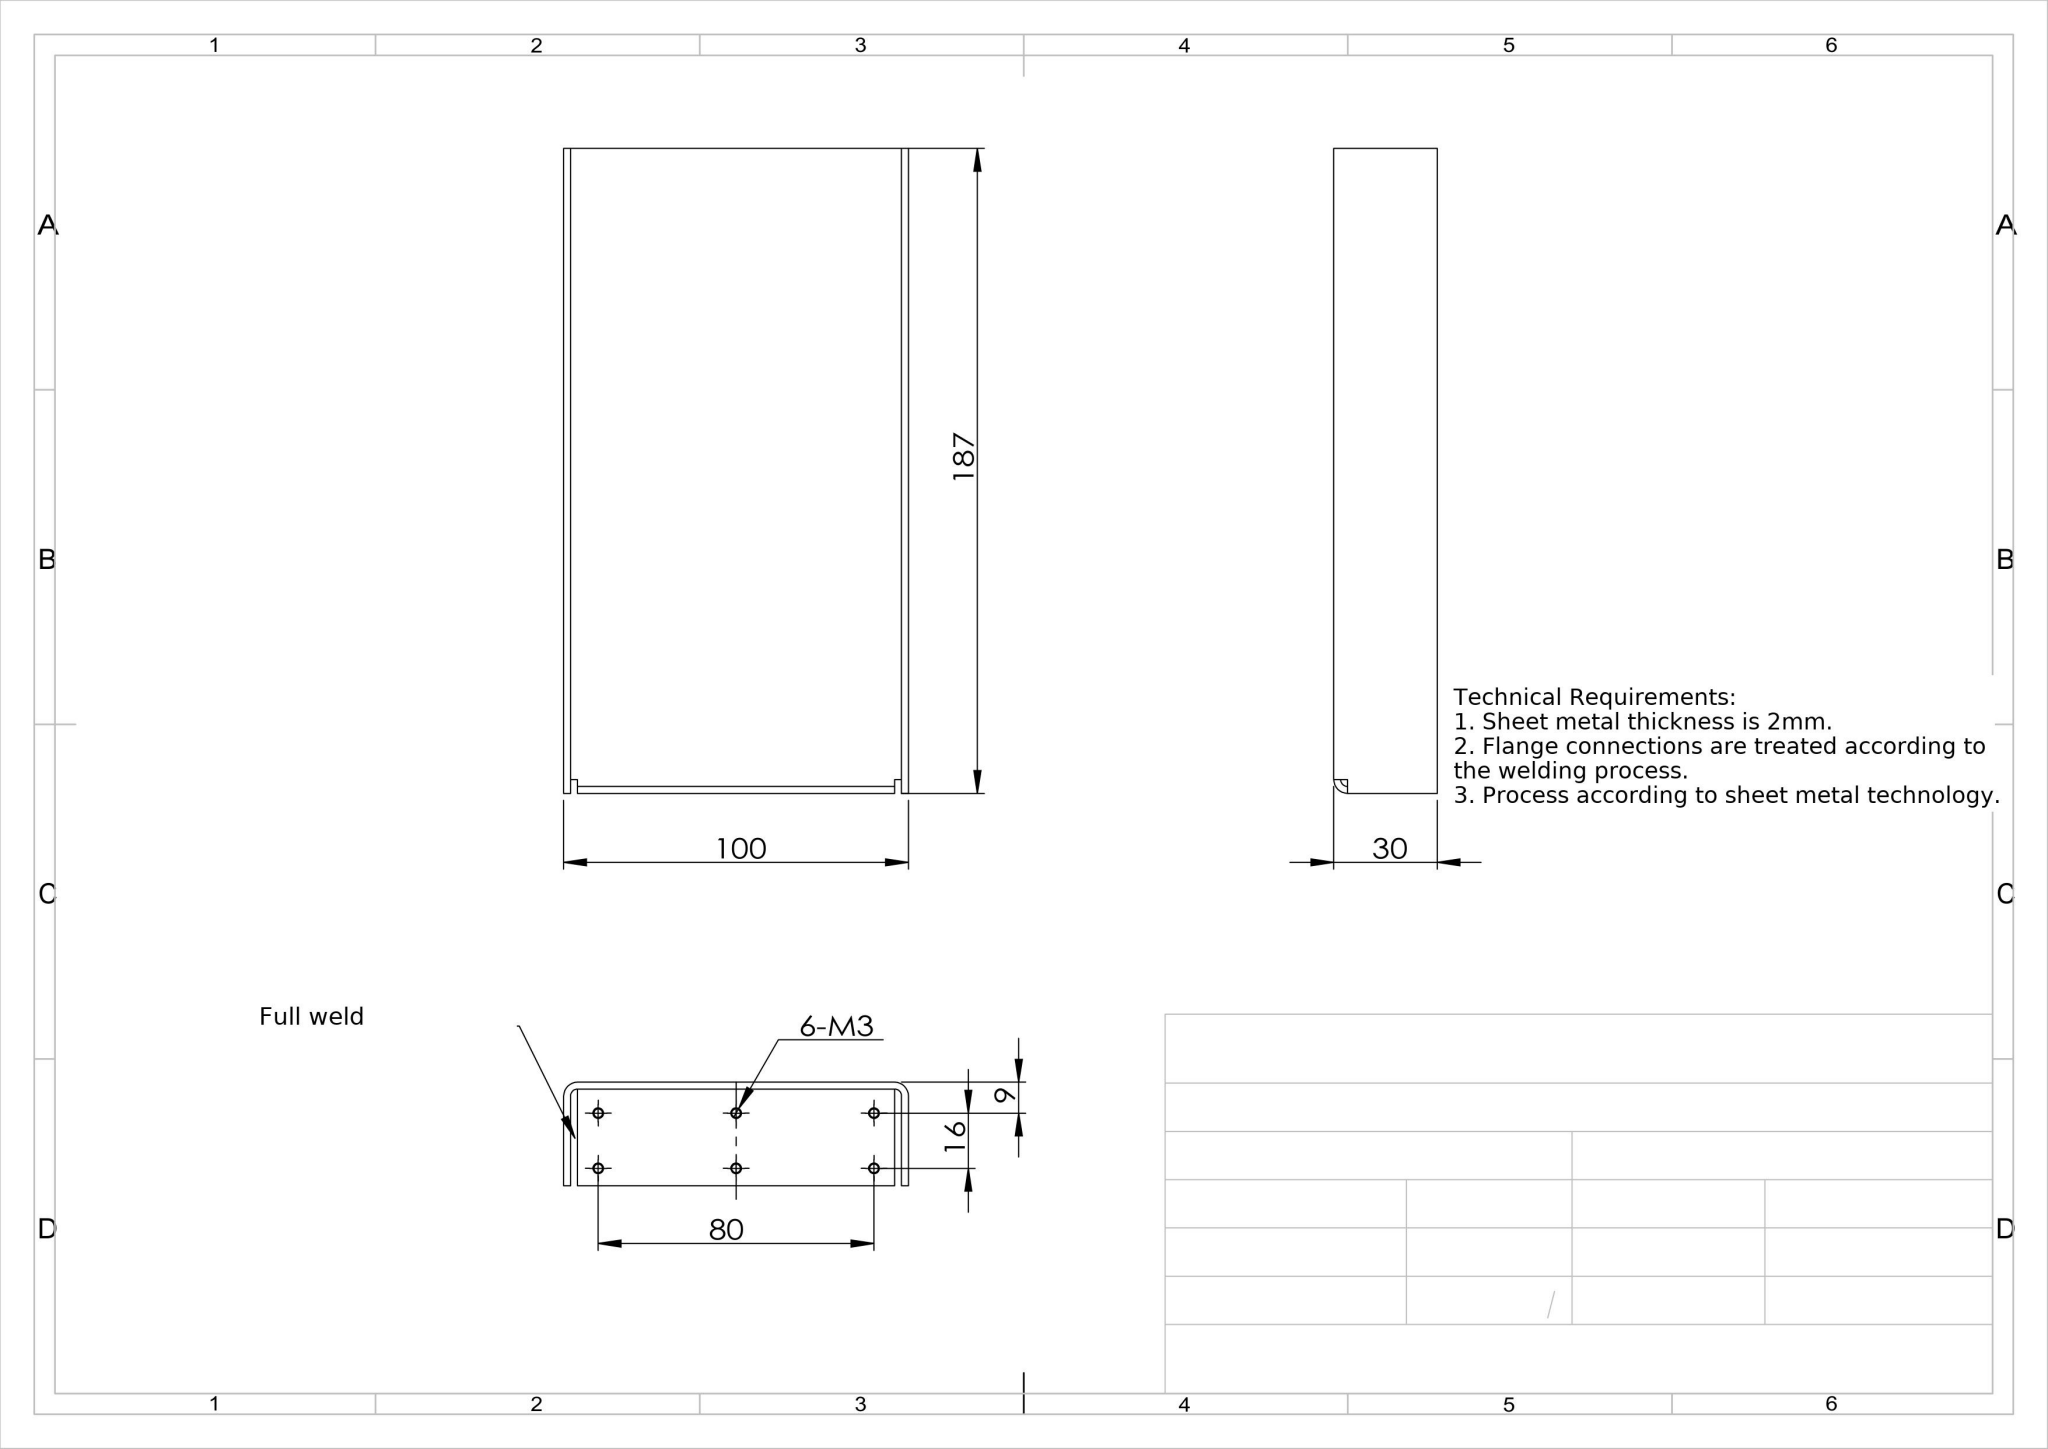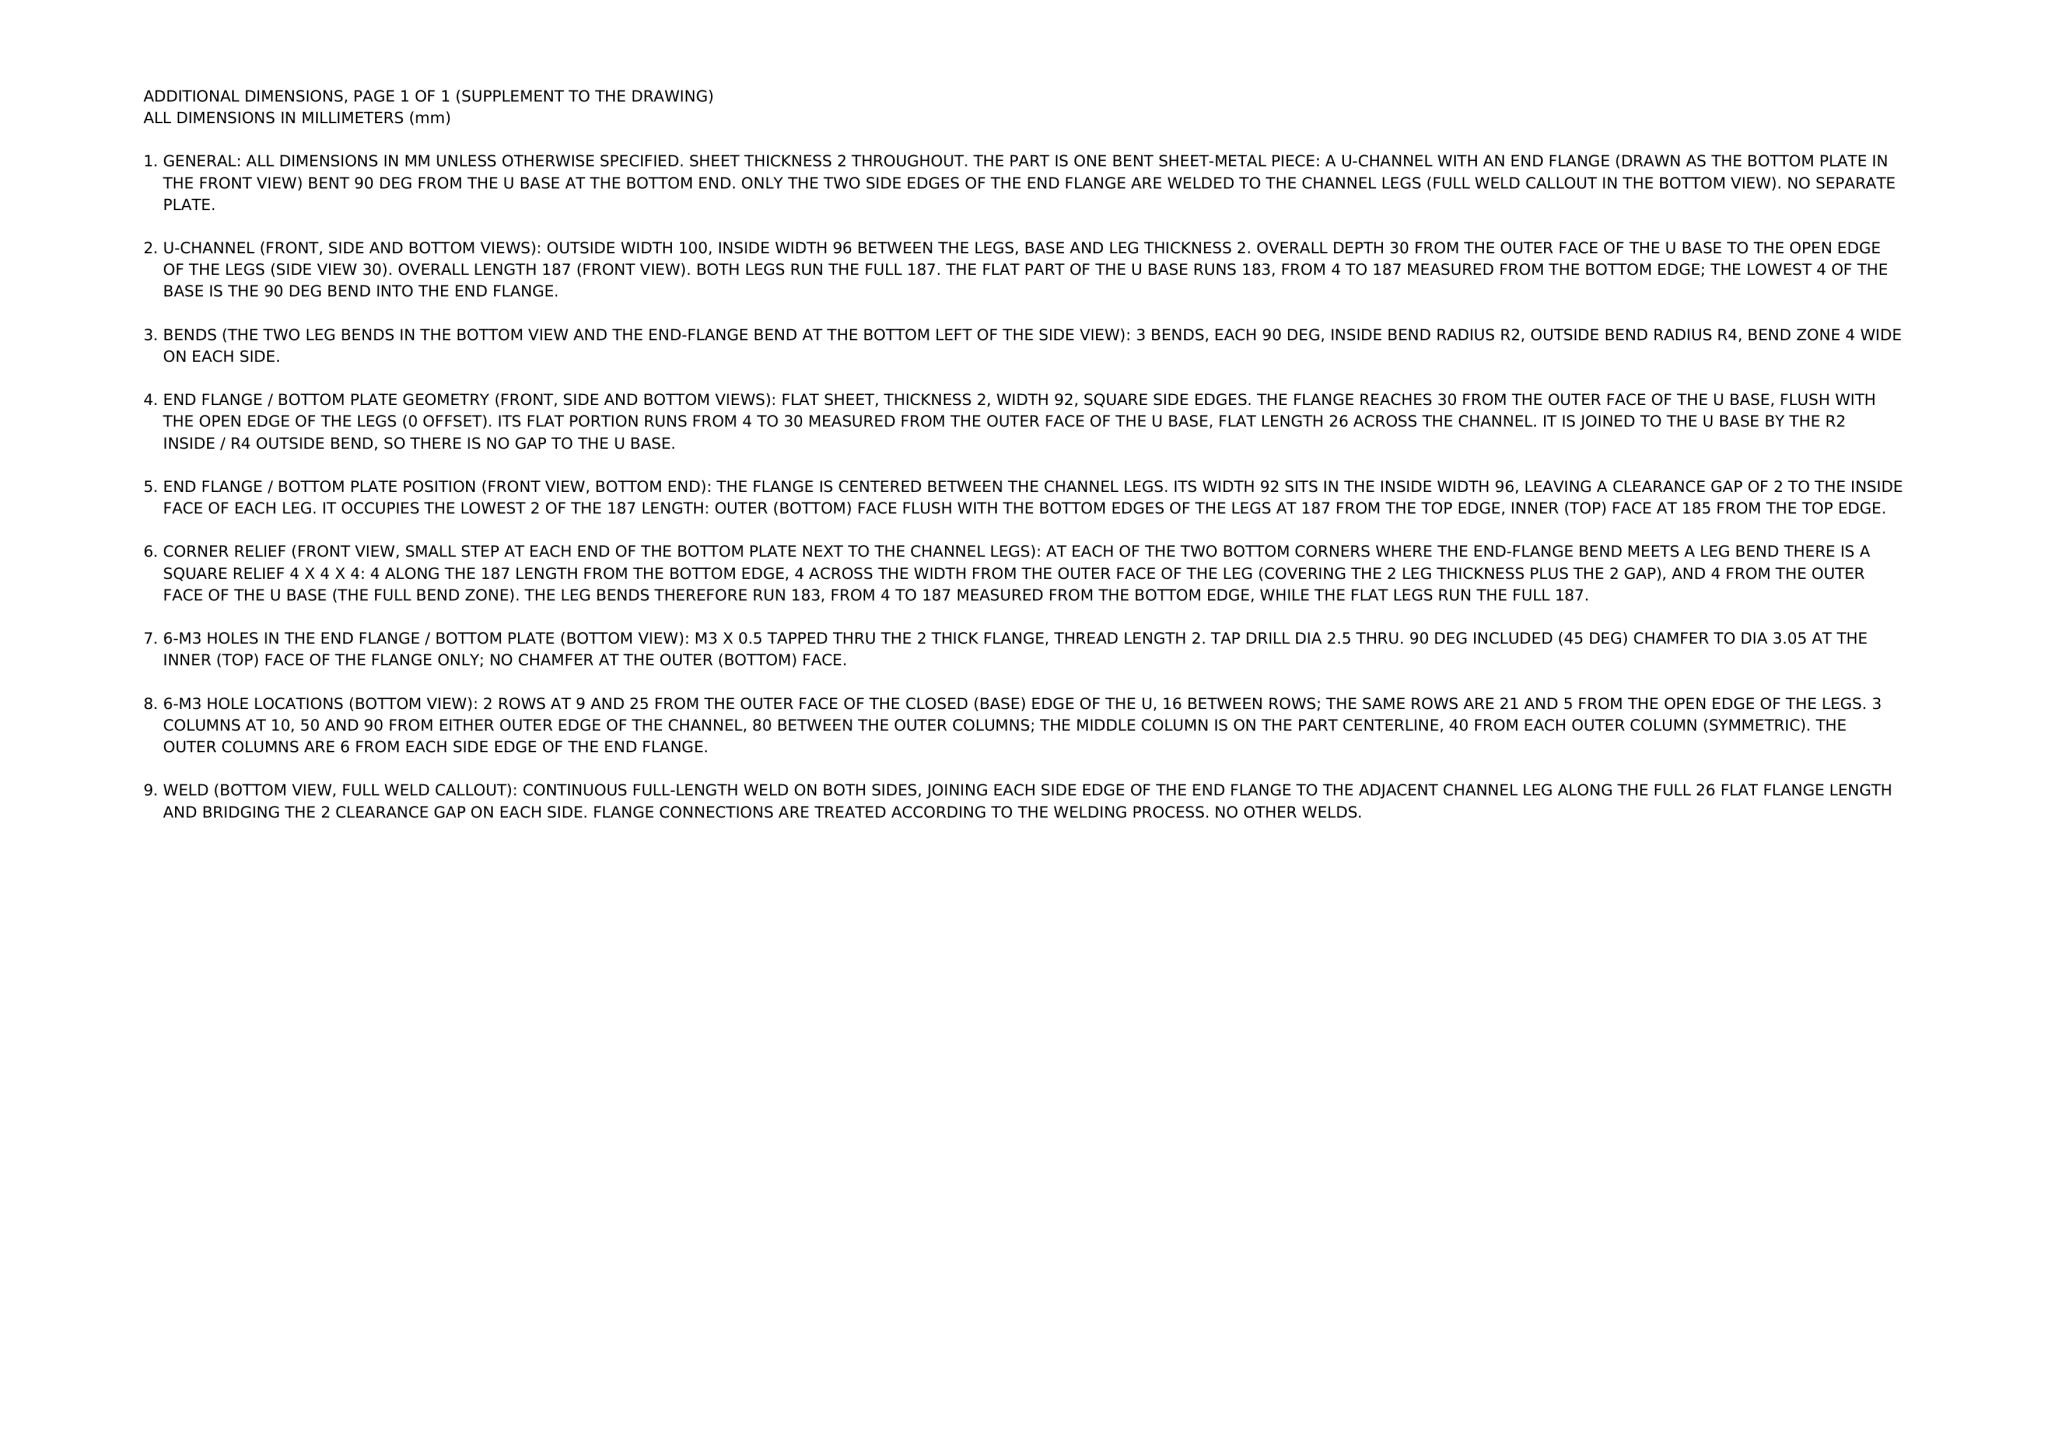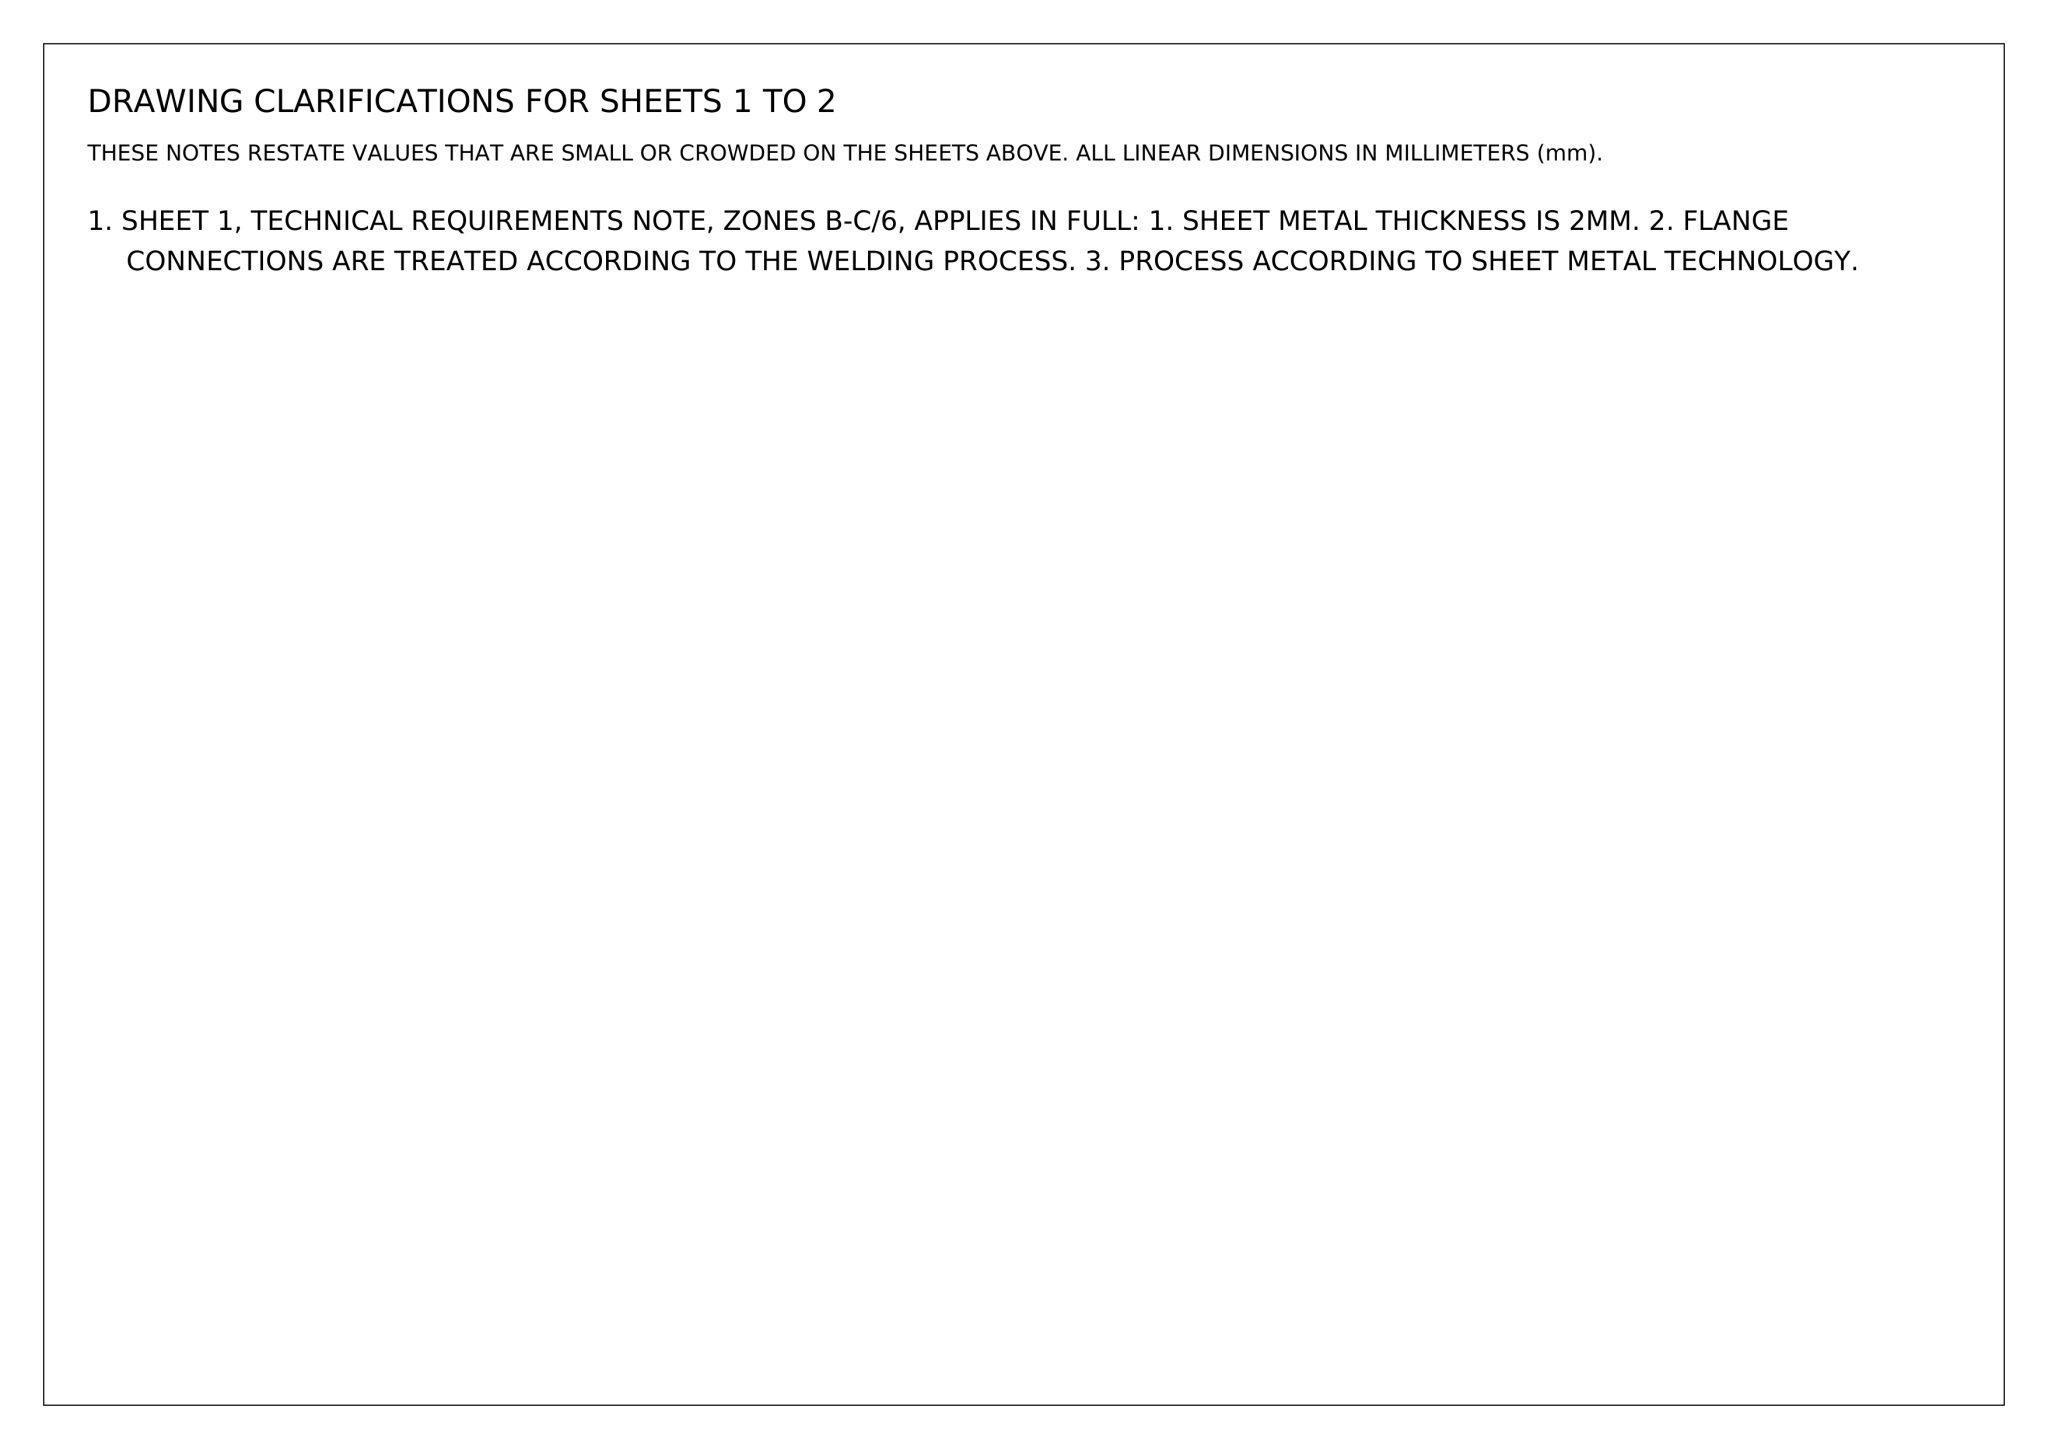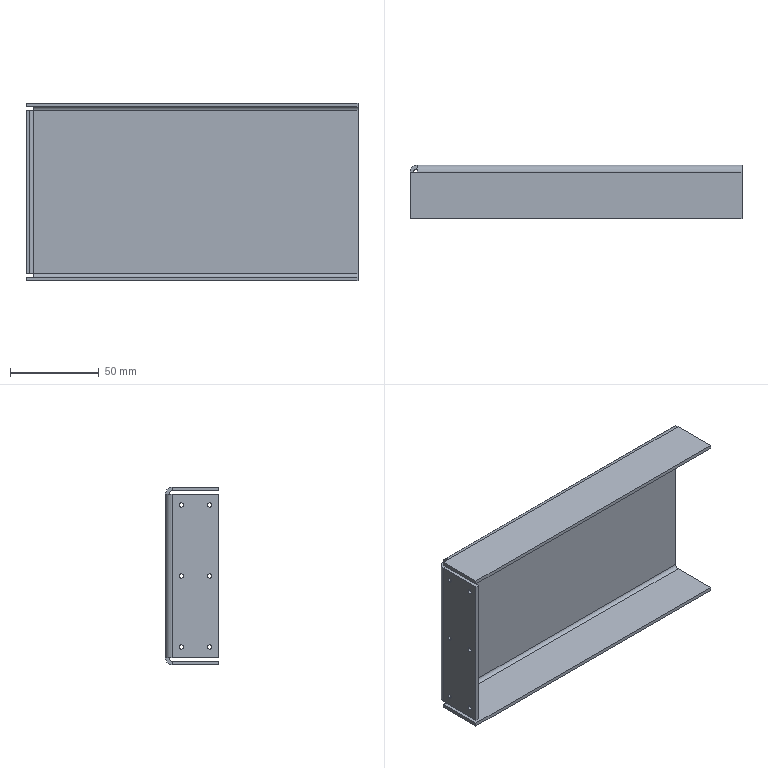Part | NX | mm | 1 solid | 56 faces | box 187 x 30 x 100 mm | volume 62160 mm3 | plane 26 | cylinder 18 | cone 12 | commonest cylinder face diameters 2.5 x12 4 x3 8 x3